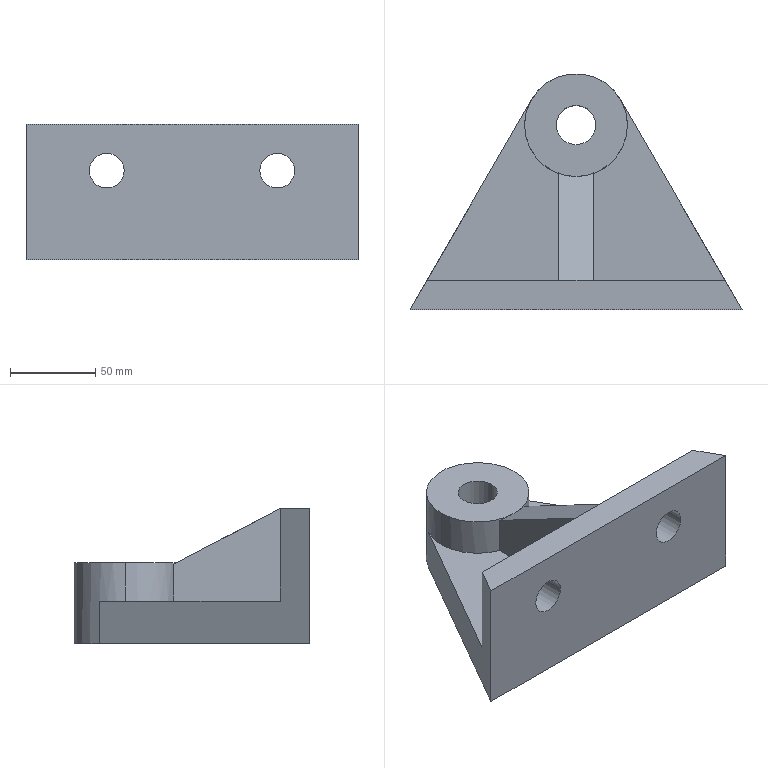Component | SolidWorks | SupportBase4-2 | 1 solid | 22 faces | box 194.91 x 138.62 x 79.5 mm | volume 650486 mm3 | plane 13 | cylinder 9 | commonest cylinder face diameters 60.351 x3 20.43 x2 20.4 x2 23 x2 | material 45
STEP:
#1=CARTESIAN_POINT('',(-2.157,-7.867,23.818));
#2=VERTEX_POINT('',#1);
#3=CARTESIAN_POINT('',(-2.961,-7.867,23.818));
#4=VERTEX_POINT('',#3);
#5=CARTESIAN_POINT('',(-2.559,-7.867,23.818));
#6=DIRECTION('',(0.,-1.,-0.));
#7=DIRECTION('',(-1.,0.,0.));
#8=AXIS2_PLACEMENT_3D('',#5,#6,#7);
#9=CIRCLE('',#8,0.4022);
#10=EDGE_CURVE('',#2,#4,#9,.T.);
#11=ORIENTED_EDGE('',*,*,#10,.T.);
#12=CARTESIAN_POINT('',(-2.961,-7.186,23.818));
#13=VERTEX_POINT('',#12);
#14=CARTESIAN_POINT('',(-2.961,-9.824,23.818));
#15=DIRECTION('',(-0.,1.,0.));
#16=VECTOR('',#15,39.37);
#17=LINE('',#14,#16);
#18=EDGE_CURVE('',#4,#13,#17,.T.);
#19=ORIENTED_EDGE('',*,*,#18,.T.);
#20=CARTESIAN_POINT('',(-2.157,-7.186,23.818));
#21=VERTEX_POINT('',#20);
#22=CARTESIAN_POINT('',(-2.559,-7.186,23.818));
#23=DIRECTION('',(-0.,1.,0.));
#24=DIRECTION('',(1.,0.,0.));
#25=AXIS2_PLACEMENT_3D('',#22,#23,#24);
#26=CIRCLE('',#25,0.4022);
#27=EDGE_CURVE('',#13,#21,#26,.T.);
#28=ORIENTED_EDGE('',*,*,#27,.T.);
#29=CARTESIAN_POINT('',(-2.157,-9.824,23.818));
#30=DIRECTION('',(-0.,1.,0.));
#31=VECTOR('',#30,39.37);
#32=LINE('',#29,#31);
#33=EDGE_CURVE('',#2,#21,#32,.T.);
#34=ORIENTED_EDGE('',*,*,#33,.F.);
#35=EDGE_LOOP('',(#11,#19,#28,#34));
#36=FACE_OUTER_BOUND('',#35,.T.);
#37=CARTESIAN_POINT('',(-2.559,-9.824,23.818));
#38=DIRECTION('',(-0.,1.,0.));
#39=DIRECTION('',(1.,0.,0.));
#40=AXIS2_PLACEMENT_3D('',#37,#38,#39);
#41=CYLINDRICAL_SURFACE('',#40,0.4022);
#42=ADVANCED_FACE('',(#36),#41,.F.);
#43=CARTESIAN_POINT('',(1.78,-7.867,23.818));
#44=VERTEX_POINT('',#43);
#45=CARTESIAN_POINT('',(0.9764,-7.867,23.818));
#46=VERTEX_POINT('',#45);
#47=CARTESIAN_POINT('',(1.378,-7.867,23.818));
#48=DIRECTION('',(0.,-1.,-0.));
#49=DIRECTION('',(-1.,0.,0.));
#50=AXIS2_PLACEMENT_3D('',#47,#48,#49);
#51=CIRCLE('',#50,0.4016);
#52=EDGE_CURVE('',#44,#46,#51,.T.);
#53=ORIENTED_EDGE('',*,*,#52,.T.);
#54=CARTESIAN_POINT('',(0.9764,-7.186,23.818));
#55=VERTEX_POINT('',#54);
#56=CARTESIAN_POINT('',(0.9764,-9.824,23.818));
#57=DIRECTION('',(-0.,1.,0.));
#58=VECTOR('',#57,39.37);
#59=LINE('',#56,#58);
#60=EDGE_CURVE('',#46,#55,#59,.T.);
#61=ORIENTED_EDGE('',*,*,#60,.T.);
#62=CARTESIAN_POINT('',(1.78,-7.186,23.818));
#63=VERTEX_POINT('',#62);
#64=CARTESIAN_POINT('',(1.378,-7.186,23.818));
#65=DIRECTION('',(-0.,1.,0.));
#66=DIRECTION('',(1.,0.,0.));
#67=AXIS2_PLACEMENT_3D('',#64,#65,#66);
#68=CIRCLE('',#67,0.4016);
#69=EDGE_CURVE('',#55,#63,#68,.T.);
#70=ORIENTED_EDGE('',*,*,#69,.T.);
#71=CARTESIAN_POINT('',(1.78,-9.824,23.818));
#72=DIRECTION('',(-0.,1.,0.));
#73=VECTOR('',#72,39.37);
#74=LINE('',#71,#73);
#75=EDGE_CURVE('',#44,#63,#74,.T.);
#76=ORIENTED_EDGE('',*,*,#75,.F.);
#77=EDGE_LOOP('',(#53,#61,#70,#76));
#78=FACE_OUTER_BOUND('',#77,.T.);
#79=CARTESIAN_POINT('',(1.378,-9.824,23.818));
#80=DIRECTION('',(-0.,1.,0.));
#81=DIRECTION('',(1.,0.,0.));
#82=AXIS2_PLACEMENT_3D('',#79,#80,#81);
#83=CYLINDRICAL_SURFACE('',#82,0.4016);
#84=ADVANCED_FACE('',(#78),#83,.F.);
#85=CARTESIAN_POINT('',(-0.1378,-3.597,21.761));
#86=VERTEX_POINT('',#85);
#87=CARTESIAN_POINT('',(-1.043,-3.597,21.761));
#88=VERTEX_POINT('',#87);
#89=CARTESIAN_POINT('',(-0.5906,-3.597,21.761));
#90=DIRECTION('',(0.,0.,-1.));
#91=DIRECTION('',(-1.,0.,0.));
#92=AXIS2_PLACEMENT_3D('',#89,#90,#91);
#93=CIRCLE('',#92,0.4528);
#94=EDGE_CURVE('',#86,#88,#93,.T.);
#95=ORIENTED_EDGE('',*,*,#94,.T.);
#96=CARTESIAN_POINT('',(-1.043,-3.597,23.631));
#97=VERTEX_POINT('',#96);
#98=CARTESIAN_POINT('',(-1.043,-3.597,21.761));
#99=DIRECTION('',(-0.,-0.,1.));
#100=VECTOR('',#99,39.37);
#101=LINE('',#98,#100);
#102=EDGE_CURVE('',#88,#97,#101,.T.);
#103=ORIENTED_EDGE('',*,*,#102,.T.);
#104=CARTESIAN_POINT('',(-0.1378,-3.597,23.631));
#105=VERTEX_POINT('',#104);
#106=CARTESIAN_POINT('',(-0.5906,-3.597,23.631));
#107=DIRECTION('',(0.,0.,-1.));
#108=DIRECTION('',(-1.,0.,0.));
#109=AXIS2_PLACEMENT_3D('',#106,#107,#108);
#110=CIRCLE('',#109,0.4528);
#111=EDGE_CURVE('',#105,#97,#110,.T.);
#112=ORIENTED_EDGE('',*,*,#111,.F.);
#113=CARTESIAN_POINT('',(-0.1378,-3.597,21.761));
#114=DIRECTION('',(-0.,-0.,1.));
#115=VECTOR('',#114,39.37);
#116=LINE('',#113,#115);
#117=EDGE_CURVE('',#86,#105,#116,.T.);
#118=ORIENTED_EDGE('',*,*,#117,.F.);
#119=EDGE_LOOP('',(#95,#103,#112,#118));
#120=FACE_OUTER_BOUND('',#119,.T.);
#121=CARTESIAN_POINT('',(-0.5906,-3.597,21.761));
#122=DIRECTION('',(-0.,-0.,1.));
#123=DIRECTION('',(1.,0.,0.));
#124=AXIS2_PLACEMENT_3D('',#121,#122,#123);
#125=CYLINDRICAL_SURFACE('',#124,0.4528);
#126=ADVANCED_FACE('',(#120),#125,.F.);
#127=CARTESIAN_POINT('',(-1.779,-3.597,22.745));
#128=VERTEX_POINT('',#127);
#129=CARTESIAN_POINT('',(-1.619,-3.003,22.745));
#130=VERTEX_POINT('',#129);
#131=CARTESIAN_POINT('',(-0.5906,-3.597,22.745));
#132=DIRECTION('',(0.,0.,-1.));
#133=DIRECTION('',(-1.,0.,0.));
#134=AXIS2_PLACEMENT_3D('',#131,#132,#133);
#135=CIRCLE('',#134,1.188);
#136=EDGE_CURVE('',#128,#130,#135,.T.);
#137=ORIENTED_EDGE('',*,*,#136,.F.);
#138=CARTESIAN_POINT('',(-1.779,-3.597,23.631));
#139=VERTEX_POINT('',#138);
#140=CARTESIAN_POINT('',(-1.779,-3.597,21.761));
#141=DIRECTION('',(-0.,-0.,1.));
#142=VECTOR('',#141,39.37);
#143=LINE('',#140,#142);
#144=EDGE_CURVE('',#128,#139,#143,.T.);
#145=ORIENTED_EDGE('',*,*,#144,.T.);
#146=CARTESIAN_POINT('',(0.5975,-3.597,23.631));
#147=VERTEX_POINT('',#146);
#148=CARTESIAN_POINT('',(-0.5906,-3.597,23.631));
#149=DIRECTION('',(0.,0.,-1.));
#150=DIRECTION('',(-1.,0.,0.));
#151=AXIS2_PLACEMENT_3D('',#148,#149,#150);
#152=CIRCLE('',#151,1.188);
#153=EDGE_CURVE('',#139,#147,#152,.T.);
#154=ORIENTED_EDGE('',*,*,#153,.T.);
#155=CARTESIAN_POINT('',(0.5975,-3.597,22.745));
#156=VERTEX_POINT('',#155);
#157=CARTESIAN_POINT('',(0.5975,-3.597,21.761));
#158=DIRECTION('',(-0.,-0.,1.));
#159=VECTOR('',#158,39.37);
#160=LINE('',#157,#159);
#161=EDGE_CURVE('',#156,#147,#160,.T.);
#162=ORIENTED_EDGE('',*,*,#161,.F.);
#163=CARTESIAN_POINT('',(0.4383,-3.003,22.745));
#164=VERTEX_POINT('',#163);
#165=CARTESIAN_POINT('',(-0.5906,-3.597,22.745));
#166=DIRECTION('',(0.,0.,-1.));
#167=DIRECTION('',(-1.,0.,0.));
#168=AXIS2_PLACEMENT_3D('',#165,#166,#167);
#169=CIRCLE('',#168,1.188);
#170=EDGE_CURVE('',#164,#156,#169,.T.);
#171=ORIENTED_EDGE('',*,*,#170,.F.);
#172=CARTESIAN_POINT('',(0.4383,-3.003,21.761));
#173=VERTEX_POINT('',#172);
#174=CARTESIAN_POINT('',(0.4383,-3.003,21.761));
#175=DIRECTION('',(-0.,-0.,1.));
#176=VECTOR('',#175,39.37);
#177=LINE('',#174,#176);
#178=EDGE_CURVE('',#173,#164,#177,.T.);
#179=ORIENTED_EDGE('',*,*,#178,.F.);
#180=CARTESIAN_POINT('',(-1.619,-3.003,21.761));
#181=VERTEX_POINT('',#180);
#182=CARTESIAN_POINT('',(-0.5906,-3.597,21.761));
#183=DIRECTION('',(0.,0.,-1.));
#184=DIRECTION('',(-1.,0.,0.));
#185=AXIS2_PLACEMENT_3D('',#182,#183,#184);
#186=CIRCLE('',#185,1.188);
#187=EDGE_CURVE('',#181,#173,#186,.T.);
#188=ORIENTED_EDGE('',*,*,#187,.F.);
#189=CARTESIAN_POINT('',(-1.619,-3.003,21.761));
#190=DIRECTION('',(-0.,-0.,1.));
#191=VECTOR('',#190,39.37);
#192=LINE('',#189,#191);
#193=EDGE_CURVE('',#181,#130,#192,.T.);
#194=ORIENTED_EDGE('',*,*,#193,.T.);
#195=EDGE_LOOP('',(#137,#145,#154,#162,#171,#179,#188,#194));
#196=FACE_OUTER_BOUND('',#195,.T.);
#197=CARTESIAN_POINT('',(-0.5906,-3.597,21.761));
#198=DIRECTION('',(-0.,-0.,1.));
#199=DIRECTION('',(1.,0.,0.));
#200=AXIS2_PLACEMENT_3D('',#197,#198,#199);
#201=CYLINDRICAL_SURFACE('',#200,1.188);
#202=ADVANCED_FACE('',(#196),#201,.T.);
#203=CARTESIAN_POINT('',(-0.1969,-4.718,22.745));
#204=VERTEX_POINT('',#203);
#205=CARTESIAN_POINT('',(-0.5906,-3.597,22.745));
#206=DIRECTION('',(0.,0.,-1.));
#207=DIRECTION('',(-1.,0.,0.));
#208=AXIS2_PLACEMENT_3D('',#205,#206,#207);
#209=CIRCLE('',#208,1.188);
#210=EDGE_CURVE('',#156,#204,#209,.T.);
#211=ORIENTED_EDGE('',*,*,#210,.F.);
#212=ORIENTED_EDGE('',*,*,#161,.T.);
#213=CARTESIAN_POINT('',(-0.5906,-4.785,23.631));
#214=VERTEX_POINT('',#213);
#215=CARTESIAN_POINT('',(-0.5906,-3.597,23.631));
#216=DIRECTION('',(0.,0.,-1.));
#217=DIRECTION('',(-1.,0.,0.));
#218=AXIS2_PLACEMENT_3D('',#215,#216,#217);
#219=CIRCLE('',#218,1.188);
#220=EDGE_CURVE('',#147,#214,#219,.T.);
#221=ORIENTED_EDGE('',*,*,#220,.T.);
#222=CARTESIAN_POINT('',(-0.1969,-4.718,23.595));
#223=VERTEX_POINT('',#222);
#224=CARTESIAN_POINT('',(-0.5906,-4.785,23.631));
#225=CARTESIAN_POINT('',(-0.4561,-4.785,23.631));
#226=CARTESIAN_POINT('',(-0.3237,-4.763,23.619));
#227=CARTESIAN_POINT('',(-0.1969,-4.718,23.595));
#228=(BOUNDED_CURVE()B_SPLINE_CURVE(3,(#224,#225,#226,#227),.UNSPECIFIED.,.F.,.F.)B_SPLINE_CURVE_WITH_KNOTS((4,4),(0.,0.3378),.UNSPECIFIED.)CURVE()GEOMETRIC_REPRESENTATION_ITEM()RATIONAL_B_SPLINE_CURVE((1.,0.9905,0.9905,1.))REPRESENTATION_ITEM(''));
#229=EDGE_CURVE('',#214,#223,#228,.T.);
#230=ORIENTED_EDGE('',*,*,#229,.T.);
#231=CARTESIAN_POINT('',(-0.1969,-4.718,21.761));
#232=DIRECTION('',(0.,0.,-1.));
#233=VECTOR('',#232,39.37);
#234=LINE('',#231,#233);
#235=EDGE_CURVE('',#223,#204,#234,.T.);
#236=ORIENTED_EDGE('',*,*,#235,.T.);
#237=EDGE_LOOP('',(#211,#212,#221,#230,#236));
#238=FACE_OUTER_BOUND('',#237,.T.);
#239=CARTESIAN_POINT('',(-0.5906,-3.597,21.761));
#240=DIRECTION('',(-0.,-0.,1.));
#241=DIRECTION('',(1.,0.,0.));
#242=AXIS2_PLACEMENT_3D('',#239,#240,#241);
#243=CYLINDRICAL_SURFACE('',#242,1.188);
#244=ADVANCED_FACE('',(#238),#243,.T.);
#245=CARTESIAN_POINT('',(-0.9843,-4.718,22.745));
#246=VERTEX_POINT('',#245);
#247=CARTESIAN_POINT('',(-0.9843,-7.186,22.745));
#248=VERTEX_POINT('',#247);
#249=CARTESIAN_POINT('',(-0.9843,-2.789,22.745));
#250=DIRECTION('',(0.,-1.,-0.));
#251=VECTOR('',#250,39.37);
#252=LINE('',#249,#251);
#253=EDGE_CURVE('',#246,#248,#252,.T.);
#254=ORIENTED_EDGE('',*,*,#253,.F.);
#255=CARTESIAN_POINT('',(-0.5906,-3.597,22.745));
#256=DIRECTION('',(0.,0.,-1.));
#257=DIRECTION('',(-1.,0.,0.));
#258=AXIS2_PLACEMENT_3D('',#255,#256,#257);
#259=CIRCLE('',#258,1.188);
#260=EDGE_CURVE('',#246,#128,#259,.T.);
#261=ORIENTED_EDGE('',*,*,#260,.T.);
#262=ORIENTED_EDGE('',*,*,#136,.T.);
#263=CARTESIAN_POINT('',(-4.034,-7.186,22.745));
#264=VERTEX_POINT('',#263);
#265=CARTESIAN_POINT('',(-1.61,-2.988,22.745));
#266=DIRECTION('',(-0.5,-0.866,-0.));
#267=VECTOR('',#266,39.37);
#268=LINE('',#265,#267);
#269=EDGE_CURVE('',#130,#264,#268,.T.);
#270=ORIENTED_EDGE('',*,*,#269,.T.);
#271=CARTESIAN_POINT('',(-1.955,-7.186,22.745));
#272=DIRECTION('',(1.,0.,0.));
#273=VECTOR('',#272,39.37);
#274=LINE('',#271,#273);
#275=EDGE_CURVE('',#264,#248,#274,.T.);
#276=ORIENTED_EDGE('',*,*,#275,.T.);
#277=EDGE_LOOP('',(#254,#261,#262,#270,#276));
#278=FACE_OUTER_BOUND('',#277,.T.);
#279=CARTESIAN_POINT('',(-1.955,-2.789,22.745));
#280=DIRECTION('',(0.,0.,-1.));
#281=DIRECTION('',(-1.,0.,-0.));
#282=AXIS2_PLACEMENT_3D('',#279,#280,#281);
#283=PLANE('',#282);
#284=ADVANCED_FACE('',(#278),#283,.F.);
#285=CARTESIAN_POINT('',(-2.559,-7.186,23.818));
#286=DIRECTION('',(-0.,1.,0.));
#287=DIRECTION('',(1.,0.,0.));
#288=AXIS2_PLACEMENT_3D('',#285,#286,#287);
#289=CIRCLE('',#288,0.4022);
#290=EDGE_CURVE('',#21,#13,#289,.T.);
#291=ORIENTED_EDGE('',*,*,#290,.F.);
#292=ORIENTED_EDGE('',*,*,#27,.F.);
#293=EDGE_LOOP('',(#291,#292));
#294=FACE_BOUND('',#293,.T.);
#295=CARTESIAN_POINT('',(-0.9843,-7.186,24.891));
#296=VERTEX_POINT('',#295);
#297=CARTESIAN_POINT('',(-0.9843,-7.186,14.057));
#298=DIRECTION('',(0.,-0.,1.));
#299=VECTOR('',#298,39.37);
#300=LINE('',#297,#299);
#301=EDGE_CURVE('',#248,#296,#300,.T.);
#302=ORIENTED_EDGE('',*,*,#301,.F.);
#303=ORIENTED_EDGE('',*,*,#275,.F.);
#304=CARTESIAN_POINT('',(-4.034,-7.186,24.891));
#305=VERTEX_POINT('',#304);
#306=CARTESIAN_POINT('',(-4.034,-7.186,14.057));
#307=DIRECTION('',(-0.,-0.,1.));
#308=VECTOR('',#307,39.37);
#309=LINE('',#306,#308);
#310=EDGE_CURVE('',#264,#305,#309,.T.);
#311=ORIENTED_EDGE('',*,*,#310,.T.);
#312=CARTESIAN_POINT('',(-1.955,-7.186,24.891));
#313=DIRECTION('',(1.,0.,0.));
#314=VECTOR('',#313,39.37);
#315=LINE('',#312,#314);
#316=EDGE_CURVE('',#305,#296,#315,.T.);
#317=ORIENTED_EDGE('',*,*,#316,.T.);
#318=EDGE_LOOP('',(#302,#303,#311,#317));
#319=FACE_OUTER_BOUND('',#318,.T.);
#320=CARTESIAN_POINT('',(-1.955,-7.186,14.057));
#321=DIRECTION('',(0.,-1.,-0.));
#322=DIRECTION('',(-1.,-0.,-0.));
#323=AXIS2_PLACEMENT_3D('',#320,#321,#322);
#324=PLANE('',#323);
#325=ADVANCED_FACE('',(#294,#319),#324,.F.);
#326=ORIENTED_EDGE('',*,*,#269,.F.);
#327=ORIENTED_EDGE('',*,*,#193,.F.);
#328=CARTESIAN_POINT('',(-4.427,-7.867,21.761));
#329=VERTEX_POINT('',#328);
#330=CARTESIAN_POINT('',(-1.61,-2.988,21.761));
#331=DIRECTION('',(-0.5,-0.866,-0.));
#332=VECTOR('',#331,39.37);
#333=LINE('',#330,#332);
#334=EDGE_CURVE('',#181,#329,#333,.T.);
#335=ORIENTED_EDGE('',*,*,#334,.T.);
#336=CARTESIAN_POINT('',(-4.427,-7.867,24.891));
#337=VERTEX_POINT('',#336);
#338=CARTESIAN_POINT('',(-4.427,-7.867,14.057));
#339=DIRECTION('',(-0.,-0.,1.));
#340=VECTOR('',#339,39.37);
#341=LINE('',#338,#340);
#342=EDGE_CURVE('',#329,#337,#341,.T.);
#343=ORIENTED_EDGE('',*,*,#342,.T.);
#344=CARTESIAN_POINT('',(-1.61,-2.988,24.891));
#345=DIRECTION('',(-0.5,-0.866,-0.));
#346=VECTOR('',#345,39.37);
#347=LINE('',#344,#346);
#348=EDGE_CURVE('',#305,#337,#347,.T.);
#349=ORIENTED_EDGE('',*,*,#348,.F.);
#350=ORIENTED_EDGE('',*,*,#310,.F.);
#351=EDGE_LOOP('',(#326,#327,#335,#343,#349,#350));
#352=FACE_OUTER_BOUND('',#351,.T.);
#353=CARTESIAN_POINT('',(-1.61,-2.988,21.761));
#354=DIRECTION('',(-0.866,0.5,0.));
#355=DIRECTION('',(0.5,0.866,0.));
#356=AXIS2_PLACEMENT_3D('',#353,#354,#355);
#357=PLANE('',#356);
#358=ADVANCED_FACE('',(#352),#357,.T.);
#359=ORIENTED_EDGE('',*,*,#144,.F.);
#360=ORIENTED_EDGE('',*,*,#260,.F.);
#361=CARTESIAN_POINT('',(-0.9843,-4.718,23.595));
#362=VERTEX_POINT('',#361);
#363=CARTESIAN_POINT('',(-0.9843,-4.718,21.761));
#364=DIRECTION('',(0.,0.,-1.));
#365=VECTOR('',#364,39.37);
#366=LINE('',#363,#365);
#367=EDGE_CURVE('',#362,#246,#366,.T.);
#368=ORIENTED_EDGE('',*,*,#367,.F.);
#369=CARTESIAN_POINT('',(-0.9843,-4.718,23.595));
#370=CARTESIAN_POINT('',(-0.8574,-4.763,23.619));
#371=CARTESIAN_POINT('',(-0.725,-4.785,23.631));
#372=CARTESIAN_POINT('',(-0.5906,-4.785,23.631));
#373=(BOUNDED_CURVE()B_SPLINE_CURVE(3,(#369,#370,#371,#372),.UNSPECIFIED.,.F.,.F.)B_SPLINE_CURVE_WITH_KNOTS((4,4),(5.945,6.283),.UNSPECIFIED.)CURVE()GEOMETRIC_REPRESENTATION_ITEM()RATIONAL_B_SPLINE_CURVE((1.,0.9905,0.9905,1.))REPRESENTATION_ITEM(''));
#374=EDGE_CURVE('',#362,#214,#373,.T.);
#375=ORIENTED_EDGE('',*,*,#374,.T.);
#376=CARTESIAN_POINT('',(-0.5906,-3.597,23.631));
#377=DIRECTION('',(0.,0.,-1.));
#378=DIRECTION('',(-1.,0.,0.));
#379=AXIS2_PLACEMENT_3D('',#376,#377,#378);
#380=CIRCLE('',#379,1.188);
#381=EDGE_CURVE('',#214,#139,#380,.T.);
#382=ORIENTED_EDGE('',*,*,#381,.T.);
#383=EDGE_LOOP('',(#359,#360,#368,#375,#382));
#384=FACE_OUTER_BOUND('',#383,.T.);
#385=CARTESIAN_POINT('',(-0.5906,-3.597,21.761));
#386=DIRECTION('',(-0.,-0.,1.));
#387=DIRECTION('',(1.,0.,0.));
#388=AXIS2_PLACEMENT_3D('',#385,#386,#387);
#389=CYLINDRICAL_SURFACE('',#388,1.188);
#390=ADVANCED_FACE('',(#384),#389,.T.);
#391=CARTESIAN_POINT('',(2.853,-7.186,22.745));
#392=VERTEX_POINT('',#391);
#393=CARTESIAN_POINT('',(-0.2528,-1.806,22.745));
#394=DIRECTION('',(0.5,-0.866,-0.));
#395=VECTOR('',#394,39.37);
#396=LINE('',#393,#395);
#397=EDGE_CURVE('',#164,#392,#396,.T.);
#398=ORIENTED_EDGE('',*,*,#397,.T.);
#399=CARTESIAN_POINT('',(2.853,-7.186,24.891));
#400=VERTEX_POINT('',#399);
#401=CARTESIAN_POINT('',(2.853,-7.186,14.057));
#402=DIRECTION('',(-0.,-0.,1.));
#403=VECTOR('',#402,39.37);
#404=LINE('',#401,#403);
#405=EDGE_CURVE('',#392,#400,#404,.T.);
#406=ORIENTED_EDGE('',*,*,#405,.T.);
#407=CARTESIAN_POINT('',(3.246,-7.867,24.891));
#408=VERTEX_POINT('',#407);
#409=CARTESIAN_POINT('',(-0.2528,-1.806,24.891));
#410=DIRECTION('',(0.5,-0.866,-0.));
#411=VECTOR('',#410,39.37);
#412=LINE('',#409,#411);
#413=EDGE_CURVE('',#400,#408,#412,.T.);
#414=ORIENTED_EDGE('',*,*,#413,.T.);
#415=CARTESIAN_POINT('',(3.246,-7.867,21.761));
#416=VERTEX_POINT('',#415);
#417=CARTESIAN_POINT('',(3.246,-7.867,14.057));
#418=DIRECTION('',(-0.,-0.,1.));
#419=VECTOR('',#418,39.37);
#420=LINE('',#417,#419);
#421=EDGE_CURVE('',#416,#408,#420,.T.);
#422=ORIENTED_EDGE('',*,*,#421,.F.);
#423=CARTESIAN_POINT('',(-0.2528,-1.806,21.761));
#424=DIRECTION('',(0.5,-0.866,-0.));
#425=VECTOR('',#424,39.37);
#426=LINE('',#423,#425);
#427=EDGE_CURVE('',#173,#416,#426,.T.);
#428=ORIENTED_EDGE('',*,*,#427,.F.);
#429=ORIENTED_EDGE('',*,*,#178,.T.);
#430=EDGE_LOOP('',(#398,#406,#414,#422,#428,#429));
#431=FACE_OUTER_BOUND('',#430,.T.);
#432=CARTESIAN_POINT('',(-0.2528,-1.806,21.761));
#433=DIRECTION('',(-0.866,-0.5,-0.));
#434=DIRECTION('',(-0.5,0.866,0.));
#435=AXIS2_PLACEMENT_3D('',#432,#433,#434);
#436=PLANE('',#435);
#437=ADVANCED_FACE('',(#431),#436,.F.);
#438=ORIENTED_EDGE('',*,*,#102,.F.);
#439=CARTESIAN_POINT('',(-0.5906,-3.597,21.761));
#440=DIRECTION('',(0.,0.,-1.));
#441=DIRECTION('',(-1.,0.,0.));
#442=AXIS2_PLACEMENT_3D('',#439,#440,#441);
#443=CIRCLE('',#442,0.4528);
#444=EDGE_CURVE('',#88,#86,#443,.T.);
#445=ORIENTED_EDGE('',*,*,#444,.T.);
#446=ORIENTED_EDGE('',*,*,#117,.T.);
#447=CARTESIAN_POINT('',(-0.5906,-3.597,23.631));
#448=DIRECTION('',(0.,0.,-1.));
#449=DIRECTION('',(-1.,0.,0.));
#450=AXIS2_PLACEMENT_3D('',#447,#448,#449);
#451=CIRCLE('',#450,0.4528);
#452=EDGE_CURVE('',#97,#105,#451,.T.);
#453=ORIENTED_EDGE('',*,*,#452,.F.);
#454=EDGE_LOOP('',(#438,#445,#446,#453));
#455=FACE_OUTER_BOUND('',#454,.T.);
#456=CARTESIAN_POINT('',(-0.5906,-3.597,21.761));
#457=DIRECTION('',(-0.,-0.,1.));
#458=DIRECTION('',(1.,0.,0.));
#459=AXIS2_PLACEMENT_3D('',#456,#457,#458);
#460=CYLINDRICAL_SURFACE('',#459,0.4528);
#461=ADVANCED_FACE('',(#455),#460,.F.);
#462=ORIENTED_EDGE('',*,*,#94,.F.);
#463=ORIENTED_EDGE('',*,*,#444,.F.);
#464=EDGE_LOOP('',(#462,#463));
#465=FACE_BOUND('',#464,.T.);
#466=ORIENTED_EDGE('',*,*,#187,.T.);
#467=ORIENTED_EDGE('',*,*,#427,.T.);
#468=CARTESIAN_POINT('',(-1.955,-7.867,21.761));
#469=DIRECTION('',(1.,0.,0.));
#470=VECTOR('',#469,39.37);
#471=LINE('',#468,#470);
#472=EDGE_CURVE('',#329,#416,#471,.T.);
#473=ORIENTED_EDGE('',*,*,#472,.F.);
#474=ORIENTED_EDGE('',*,*,#334,.F.);
#475=EDGE_LOOP('',(#466,#467,#473,#474));
#476=FACE_OUTER_BOUND('',#475,.T.);
#477=CARTESIAN_POINT('',(-1.955,-2.789,21.761));
#478=DIRECTION('',(0.,0.,-1.));
#479=DIRECTION('',(-1.,0.,-0.));
#480=AXIS2_PLACEMENT_3D('',#477,#478,#479);
#481=PLANE('',#480);
#482=ADVANCED_FACE('',(#465,#476),#481,.T.);
#483=ORIENTED_EDGE('',*,*,#170,.T.);
#484=ORIENTED_EDGE('',*,*,#210,.T.);
#485=CARTESIAN_POINT('',(-0.1969,-7.186,22.745));
#486=VERTEX_POINT('',#485);
#487=CARTESIAN_POINT('',(-0.1969,-2.789,22.745));
#488=DIRECTION('',(0.,-1.,-0.));
#489=VECTOR('',#488,39.37);
#490=LINE('',#487,#489);
#491=EDGE_CURVE('',#204,#486,#490,.T.);
#492=ORIENTED_EDGE('',*,*,#491,.T.);
#493=CARTESIAN_POINT('',(-1.955,-7.186,22.745));
#494=DIRECTION('',(1.,0.,0.));
#495=VECTOR('',#494,39.37);
#496=LINE('',#493,#495);
#497=EDGE_CURVE('',#486,#392,#496,.T.);
#498=ORIENTED_EDGE('',*,*,#497,.T.);
#499=ORIENTED_EDGE('',*,*,#397,.F.);
#500=EDGE_LOOP('',(#483,#484,#492,#498,#499));
#501=FACE_OUTER_BOUND('',#500,.T.);
#502=CARTESIAN_POINT('',(-1.955,-2.789,22.745));
#503=DIRECTION('',(0.,0.,-1.));
#504=DIRECTION('',(-1.,0.,-0.));
#505=AXIS2_PLACEMENT_3D('',#502,#503,#504);
#506=PLANE('',#505);
#507=ADVANCED_FACE('',(#501),#506,.F.);
#508=ORIENTED_EDGE('',*,*,#421,.T.);
#509=CARTESIAN_POINT('',(-1.955,-7.867,24.891));
#510=DIRECTION('',(1.,0.,0.));
#511=VECTOR('',#510,39.37);
#512=LINE('',#509,#511);
#513=EDGE_CURVE('',#337,#408,#512,.T.);
#514=ORIENTED_EDGE('',*,*,#513,.F.);
#515=ORIENTED_EDGE('',*,*,#342,.F.);
#516=ORIENTED_EDGE('',*,*,#472,.T.);
#517=EDGE_LOOP('',(#508,#514,#515,#516));
#518=FACE_OUTER_BOUND('',#517,.T.);
#519=ORIENTED_EDGE('',*,*,#52,.F.);
#520=CARTESIAN_POINT('',(1.378,-7.867,23.818));
#521=DIRECTION('',(0.,-1.,-0.));
#522=DIRECTION('',(-1.,0.,0.));
#523=AXIS2_PLACEMENT_3D('',#520,#521,#522);
#524=CIRCLE('',#523,0.4016);
#525=EDGE_CURVE('',#46,#44,#524,.T.);
#526=ORIENTED_EDGE('',*,*,#525,.F.);
#527=EDGE_LOOP('',(#519,#526));
#528=FACE_BOUND('',#527,.T.);
#529=ORIENTED_EDGE('',*,*,#10,.F.);
#530=CARTESIAN_POINT('',(-2.559,-7.867,23.818));
#531=DIRECTION('',(0.,-1.,-0.));
#532=DIRECTION('',(-1.,0.,0.));
#533=AXIS2_PLACEMENT_3D('',#530,#531,#532);
#534=CIRCLE('',#533,0.4022);
#535=EDGE_CURVE('',#4,#2,#534,.T.);
#536=ORIENTED_EDGE('',*,*,#535,.F.);
#537=EDGE_LOOP('',(#529,#536));
#538=FACE_BOUND('',#537,.T.);
#539=CARTESIAN_POINT('',(-1.955,-7.867,14.057));
#540=DIRECTION('',(0.,-1.,-0.));
#541=DIRECTION('',(-1.,-0.,-0.));
#542=AXIS2_PLACEMENT_3D('',#539,#540,#541);
#543=PLANE('',#542);
#544=ADVANCED_FACE('',(#518,#528,#538),#543,.T.);
#545=CARTESIAN_POINT('',(1.378,-7.186,23.818));
#546=DIRECTION('',(-0.,1.,0.));
#547=DIRECTION('',(1.,0.,0.));
#548=AXIS2_PLACEMENT_3D('',#545,#546,#547);
#549=CIRCLE('',#548,0.4016);
#550=EDGE_CURVE('',#63,#55,#549,.T.);
#551=ORIENTED_EDGE('',*,*,#550,.F.);
#552=ORIENTED_EDGE('',*,*,#69,.F.);
#553=EDGE_LOOP('',(#551,#552));
#554=FACE_BOUND('',#553,.T.);
#555=ORIENTED_EDGE('',*,*,#497,.F.);
#556=CARTESIAN_POINT('',(-0.1969,-7.186,24.891));
#557=VERTEX_POINT('',#556);
#558=CARTESIAN_POINT('',(-0.1969,-7.186,14.057));
#559=DIRECTION('',(0.,-0.,1.));
#560=VECTOR('',#559,39.37);
#561=LINE('',#558,#560);
#562=EDGE_CURVE('',#486,#557,#561,.T.);
#563=ORIENTED_EDGE('',*,*,#562,.T.);
#564=CARTESIAN_POINT('',(-1.955,-7.186,24.891));
#565=DIRECTION('',(1.,0.,0.));
#566=VECTOR('',#565,39.37);
#567=LINE('',#564,#566);
#568=EDGE_CURVE('',#557,#400,#567,.T.);
#569=ORIENTED_EDGE('',*,*,#568,.T.);
#570=ORIENTED_EDGE('',*,*,#405,.F.);
#571=EDGE_LOOP('',(#555,#563,#569,#570));
#572=FACE_OUTER_BOUND('',#571,.T.);
#573=CARTESIAN_POINT('',(-1.955,-7.186,14.057));
#574=DIRECTION('',(0.,-1.,-0.));
#575=DIRECTION('',(-1.,-0.,-0.));
#576=AXIS2_PLACEMENT_3D('',#573,#574,#575);
#577=PLANE('',#576);
#578=ADVANCED_FACE('',(#554,#572),#577,.F.);
#579=ORIENTED_EDGE('',*,*,#568,.F.);
#580=CARTESIAN_POINT('',(-1.955,-7.186,24.891));
#581=DIRECTION('',(1.,-0.,0.));
#582=VECTOR('',#581,39.37);
#583=LINE('',#580,#582);
#584=EDGE_CURVE('',#296,#557,#583,.T.);
#585=ORIENTED_EDGE('',*,*,#584,.F.);
#586=ORIENTED_EDGE('',*,*,#316,.F.);
#587=ORIENTED_EDGE('',*,*,#348,.T.);
#588=ORIENTED_EDGE('',*,*,#513,.T.);
#589=ORIENTED_EDGE('',*,*,#413,.F.);
#590=EDGE_LOOP('',(#579,#585,#586,#587,#588,#589));
#591=FACE_OUTER_BOUND('',#590,.T.);
#592=CARTESIAN_POINT('',(-1.955,-2.789,24.891));
#593=DIRECTION('',(0.,0.,-1.));
#594=DIRECTION('',(-1.,0.,-0.));
#595=AXIS2_PLACEMENT_3D('',#592,#593,#594);
#596=PLANE('',#595);
#597=ADVANCED_FACE('',(#591),#596,.F.);
#598=ORIENTED_EDGE('',*,*,#60,.F.);
#599=ORIENTED_EDGE('',*,*,#525,.T.);
#600=ORIENTED_EDGE('',*,*,#75,.T.);
#601=ORIENTED_EDGE('',*,*,#550,.T.);
#602=EDGE_LOOP('',(#598,#599,#600,#601));
#603=FACE_OUTER_BOUND('',#602,.T.);
#604=CARTESIAN_POINT('',(1.378,-9.824,23.818));
#605=DIRECTION('',(-0.,1.,0.));
#606=DIRECTION('',(1.,0.,0.));
#607=AXIS2_PLACEMENT_3D('',#604,#605,#606);
#608=CYLINDRICAL_SURFACE('',#607,0.4016);
#609=ADVANCED_FACE('',(#603),#608,.F.);
#610=ORIENTED_EDGE('',*,*,#18,.F.);
#611=ORIENTED_EDGE('',*,*,#535,.T.);
#612=ORIENTED_EDGE('',*,*,#33,.T.);
#613=ORIENTED_EDGE('',*,*,#290,.T.);
#614=EDGE_LOOP('',(#610,#611,#612,#613));
#615=FACE_OUTER_BOUND('',#614,.T.);
#616=CARTESIAN_POINT('',(-2.559,-9.824,23.818));
#617=DIRECTION('',(-0.,1.,0.));
#618=DIRECTION('',(1.,0.,0.));
#619=AXIS2_PLACEMENT_3D('',#616,#617,#618);
#620=CYLINDRICAL_SURFACE('',#619,0.4022);
#621=ADVANCED_FACE('',(#615),#620,.F.);
#622=ORIENTED_EDGE('',*,*,#111,.T.);
#623=ORIENTED_EDGE('',*,*,#452,.T.);
#624=EDGE_LOOP('',(#622,#623));
#625=FACE_BOUND('',#624,.T.);
#626=ORIENTED_EDGE('',*,*,#381,.F.);
#627=ORIENTED_EDGE('',*,*,#220,.F.);
#628=ORIENTED_EDGE('',*,*,#153,.F.);
#629=EDGE_LOOP('',(#626,#627,#628));
#630=FACE_OUTER_BOUND('',#629,.T.);
#631=CARTESIAN_POINT('',(-1.955,-2.789,23.631));
#632=DIRECTION('',(0.,0.,-1.));
#633=DIRECTION('',(-1.,0.,-0.));
#634=AXIS2_PLACEMENT_3D('',#631,#632,#633);
#635=PLANE('',#634);
#636=ADVANCED_FACE('',(#625,#630),#635,.F.);
#637=ORIENTED_EDGE('',*,*,#235,.F.);
#638=CARTESIAN_POINT('',(-0.1969,-4.785,23.631));
#639=DIRECTION('',(-0.,-0.8855,0.4647));
#640=VECTOR('',#639,39.37);
#641=LINE('',#638,#640);
#642=EDGE_CURVE('',#223,#557,#641,.T.);
#643=ORIENTED_EDGE('',*,*,#642,.T.);
#644=ORIENTED_EDGE('',*,*,#562,.F.);
#645=ORIENTED_EDGE('',*,*,#491,.F.);
#646=EDGE_LOOP('',(#637,#643,#644,#645));
#647=FACE_OUTER_BOUND('',#646,.T.);
#648=CARTESIAN_POINT('',(-0.1969,-5.138,23.326));
#649=DIRECTION('',(1.,0.,-0.));
#650=DIRECTION('',(-0.,0.,-1.));
#651=AXIS2_PLACEMENT_3D('',#648,#649,#650);
#652=PLANE('',#651);
#653=ADVANCED_FACE('',(#647),#652,.T.);
#654=CARTESIAN_POINT('',(-0.9843,-4.785,23.631));
#655=DIRECTION('',(-0.,-0.8855,0.4647));
#656=VECTOR('',#655,39.37);
#657=LINE('',#654,#656);
#658=EDGE_CURVE('',#362,#296,#657,.T.);
#659=ORIENTED_EDGE('',*,*,#658,.F.);
#660=ORIENTED_EDGE('',*,*,#367,.T.);
#661=ORIENTED_EDGE('',*,*,#253,.T.);
#662=ORIENTED_EDGE('',*,*,#301,.T.);
#663=EDGE_LOOP('',(#659,#660,#661,#662));
#664=FACE_OUTER_BOUND('',#663,.T.);
#665=CARTESIAN_POINT('',(-0.9843,-5.138,23.326));
#666=DIRECTION('',(1.,0.,-0.));
#667=DIRECTION('',(-0.,0.,-1.));
#668=AXIS2_PLACEMENT_3D('',#665,#666,#667);
#669=PLANE('',#668);
#670=ADVANCED_FACE('',(#664),#669,.F.);
#671=ORIENTED_EDGE('',*,*,#229,.F.);
#672=ORIENTED_EDGE('',*,*,#374,.F.);
#673=ORIENTED_EDGE('',*,*,#658,.T.);
#674=ORIENTED_EDGE('',*,*,#584,.T.);
#675=ORIENTED_EDGE('',*,*,#642,.F.);
#676=EDGE_LOOP('',(#671,#672,#673,#674,#675));
#677=FACE_OUTER_BOUND('',#676,.T.);
#678=CARTESIAN_POINT('',(-0.5906,-4.785,23.631));
#679=DIRECTION('',(0.,0.4647,0.8855));
#680=DIRECTION('',(-0.,-0.8855,0.4647));
#681=AXIS2_PLACEMENT_3D('',#678,#679,#680);
#682=PLANE('',#681);
#683=ADVANCED_FACE('',(#677),#682,.T.);
#684=CLOSED_SHELL('',(#42,#84,#126,#202,#244,#284,#325,#358,#390,#437,#461,#482,#507,#544,#578,#597,#609,#621,#636,#653,#670,#683));
#685=MANIFOLD_SOLID_BREP('',#684);
#686=CARTESIAN_POINT('',(0.,0.,0.));
#687=DIRECTION('',(0.,0.,1.));
#688=DIRECTION('',(1.,0.,0.));
#689=AXIS2_PLACEMENT_3D('',#686,#687,#688);
#690=(LENGTH_UNIT()NAMED_UNIT(*)SI_UNIT($,.METRE.));
#691=LENGTH_MEASURE_WITH_UNIT(LENGTH_MEASURE(0.0254),#690);
#692=DIMENSIONAL_EXPONENTS(1.,0.,0.,0.,0.,0.,0.);
#693=(CONVERSION_BASED_UNIT('',#691)LENGTH_UNIT()NAMED_UNIT(#692));
#694=UNCERTAINTY_MEASURE_WITH_UNIT(LENGTH_MEASURE(0.00001),#693,'','');
#695=(NAMED_UNIT(*)PLANE_ANGLE_UNIT()SI_UNIT($,.RADIAN.));
#696=(NAMED_UNIT(*)SI_UNIT($,.STERADIAN.)SOLID_ANGLE_UNIT());
#697=(GEOMETRIC_REPRESENTATION_CONTEXT(3)GLOBAL_UNCERTAINTY_ASSIGNED_CONTEXT((#694))GLOBAL_UNIT_ASSIGNED_CONTEXT((#693,#695,#696))REPRESENTATION_CONTEXT('',''));
#698=ADVANCED_BREP_SHAPE_REPRESENTATION('',(#685,#689),#697);
#699=COLOUR_RGB('',0.7922,0.8196,0.9333);
#700=FILL_AREA_STYLE_COLOUR('',#699);
#701=FILL_AREA_STYLE('',(#700));
#702=SURFACE_STYLE_FILL_AREA(#701);
#703=SURFACE_SIDE_STYLE('',(#702));
#704=SURFACE_STYLE_USAGE(.BOTH.,#703);
#705=PRESENTATION_STYLE_ASSIGNMENT((#704));
#706=STYLED_ITEM('',(#705),#685);
#707=(LENGTH_UNIT()NAMED_UNIT(*)SI_UNIT($,.METRE.));
#708=LENGTH_MEASURE_WITH_UNIT(LENGTH_MEASURE(0.0254),#707);
#709=DIMENSIONAL_EXPONENTS(1.,0.,0.,0.,0.,0.,0.);
#710=(CONVERSION_BASED_UNIT('',#708)LENGTH_UNIT()NAMED_UNIT(#709));
#711=UNCERTAINTY_MEASURE_WITH_UNIT(LENGTH_MEASURE(0.00001),#710,'','');
#712=(NAMED_UNIT(*)PLANE_ANGLE_UNIT()SI_UNIT($,.RADIAN.));
#713=(NAMED_UNIT(*)SI_UNIT($,.STERADIAN.)SOLID_ANGLE_UNIT());
#714=(GEOMETRIC_REPRESENTATION_CONTEXT(3)GLOBAL_UNCERTAINTY_ASSIGNED_CONTEXT((#711))GLOBAL_UNIT_ASSIGNED_CONTEXT((#710,#712,#713))REPRESENTATION_CONTEXT('',''));
#715=MECHANICAL_DESIGN_GEOMETRIC_PRESENTATION_REPRESENTATION('',(#706),#714);
#716=PRESENTATION_LAYER_ASSIGNMENT('','',(#706));